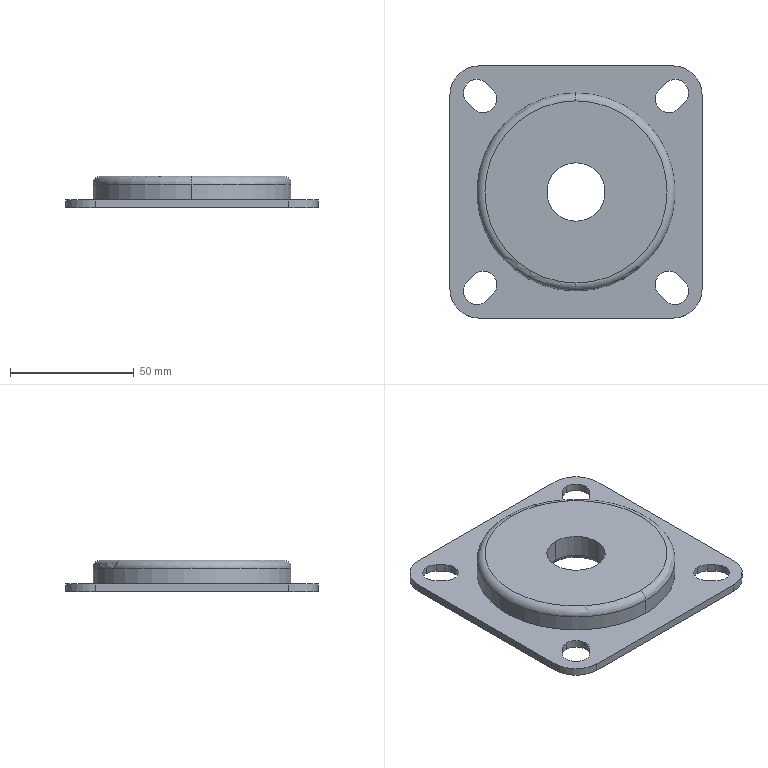Component | SolidWorks | CMAS50_F-2_CMAS50_Fswivel-1 | 1 solid | 44 faces | box 102 x 102 x 12.8 mm | volume 67826 mm3 | cylinder 22 | plane 16 | torus 6 | commonest cylinder face diameters 11 x12 24 x4 23.6 x2 80 x2 70 x2 | material 45
build123d program:
from build123d import *

# Parameters (mm, degrees)
EXTRUDE1_DEPTH = 3.2


with BuildPart() as part:
    # Sketch1 → Extrude1 (new body)
    with BuildSketch(Plane(origin=(0, 0, 0), x_dir=(1, 0, 0), z_dir=(0, 1, 0))):
        with BuildLine():
            Line((-51, 39), (-51, -39))
            ThreePointArc((-51, -39), (-47.485, -47.485), (-39, -51))
            Line((-39, -51), (39, -51))
            ThreePointArc((39, -51), (47.485, -47.485), (51, -39))
            Line((51, -39), (51, 39))
            ThreePointArc((51, 39), (47.485, 47.485), (39, 51))
            Line((39, 51), (-39, 51))
            ThreePointArc((-39, 51), (-47.485, 47.485), (-51, 39))
        make_face()
        with BuildLine():
            Line((33.611, -41.389), (36.111, -43.889))
            ThreePointArc((36.111, -43.889), (43.889, -43.889), (43.889, -36.111))
            Line((43.889, -36.111), (41.389, -33.611))
            ThreePointArc((41.389, -33.611), (33.611, -33.611), (33.611, -41.389))
        make_face(mode=Mode.SUBTRACT)
        with BuildLine():
            Line((41.389, 33.611), (43.889, 36.111))
            ThreePointArc((43.889, 36.111), (43.889, 43.889), (36.111, 43.889))
            Line((36.111, 43.889), (33.611, 41.389))
            ThreePointArc((33.611, 41.389), (33.611, 33.611), (41.389, 33.611))
        make_face(mode=Mode.SUBTRACT)
        with BuildLine():
            Line((-36.111, -43.889), (-33.611, -41.389))
            ThreePointArc((-33.611, -41.389), (-33.611, -33.611), (-41.389, -33.611))
            Line((-41.389, -33.611), (-43.889, -36.111))
            ThreePointArc((-43.889, -36.111), (-43.889, -43.889), (-36.111, -43.889))
        make_face(mode=Mode.SUBTRACT)
        with BuildLine():
            Line((-43.889, 36.111), (-41.389, 33.611))
            ThreePointArc((-41.389, 33.611), (-33.611, 33.611), (-33.611, 41.389))
            Line((-33.611, 41.389), (-36.111, 43.889))
            ThreePointArc((-36.111, 43.889), (-43.889, 43.889), (-43.889, 36.111))
        make_face(mode=Mode.SUBTRACT)
    extrude(amount=-EXTRUDE1_DEPTH)

    # Sketch2 → Cut-Revolve1 (revolve, cut)
    with BuildSketch(Plane.XY, mode=Mode.PRIVATE) as cut_revolve1_sk:
        with BuildLine():
            Line((0, 0), (35, 0))
            Line((35, 0), (35, -0.5333))
            ThreePointArc((35, -0.5333), (34.688, -1.288), (33.933, -1.6))
            Line((33.933, -1.6), (0, -1.6))
            Line((0, -1.6), (0, 0))
        make_face()
    revolve(cut_revolve1_sk.sketch.rotate(Axis((0, -1.6, 0), (0, 1, 0)), 270), axis=Axis((0, -1.6, 0), (0, 1, 0)), mode=Mode.SUBTRACT)

    # Sketch3 → Revolve1 (revolve)
    with BuildSketch(Plane.XY, mode=Mode.PRIVATE) as revolve1_sk:
        with BuildLine():
            Line((0, -3.2), (40, -3.2))
            Line((40, -3.2), (40, -9.6))
            ThreePointArc((40, -9.6), (39.063, -11.863), (36.8, -12.8))
            Line((36.8, -12.8), (0, -12.8))
            Line((0, -12.8), (0, -3.2))
        make_face()
    revolve(revolve1_sk.sketch.rotate(Axis((0, -12.8, 0), (0, 1, 0)), 270), axis=Axis((0, -12.8, 0), (0, 1, 0)))

    # Sketch4 → Cut-Revolve2 (revolve, cut)
    with BuildSketch(Plane.XY, mode=Mode.PRIVATE) as cut_revolve2_sk:
        with BuildLine():
            Line((0, -1.6), (13.8, -1.6))
            ThreePointArc((13.8, -1.6), (12.386, -2.186), (11.8, -3.6))
            Line((11.8, -3.6), (11.8, -12.8))
            Line((11.8, -12.8), (0, -12.8))
            Line((0, -12.8), (0, -1.6))
        make_face()
    revolve(cut_revolve2_sk.sketch.rotate(Axis((0, -12.8, 0), (0, 1, 0)), 270), axis=Axis((0, -12.8, 0), (0, 1, 0)), mode=Mode.SUBTRACT)


solid = part.part

# Placed as in the assembly
solid = solid.moved(Location((264, 559, 620), (-90, 0, 0)))